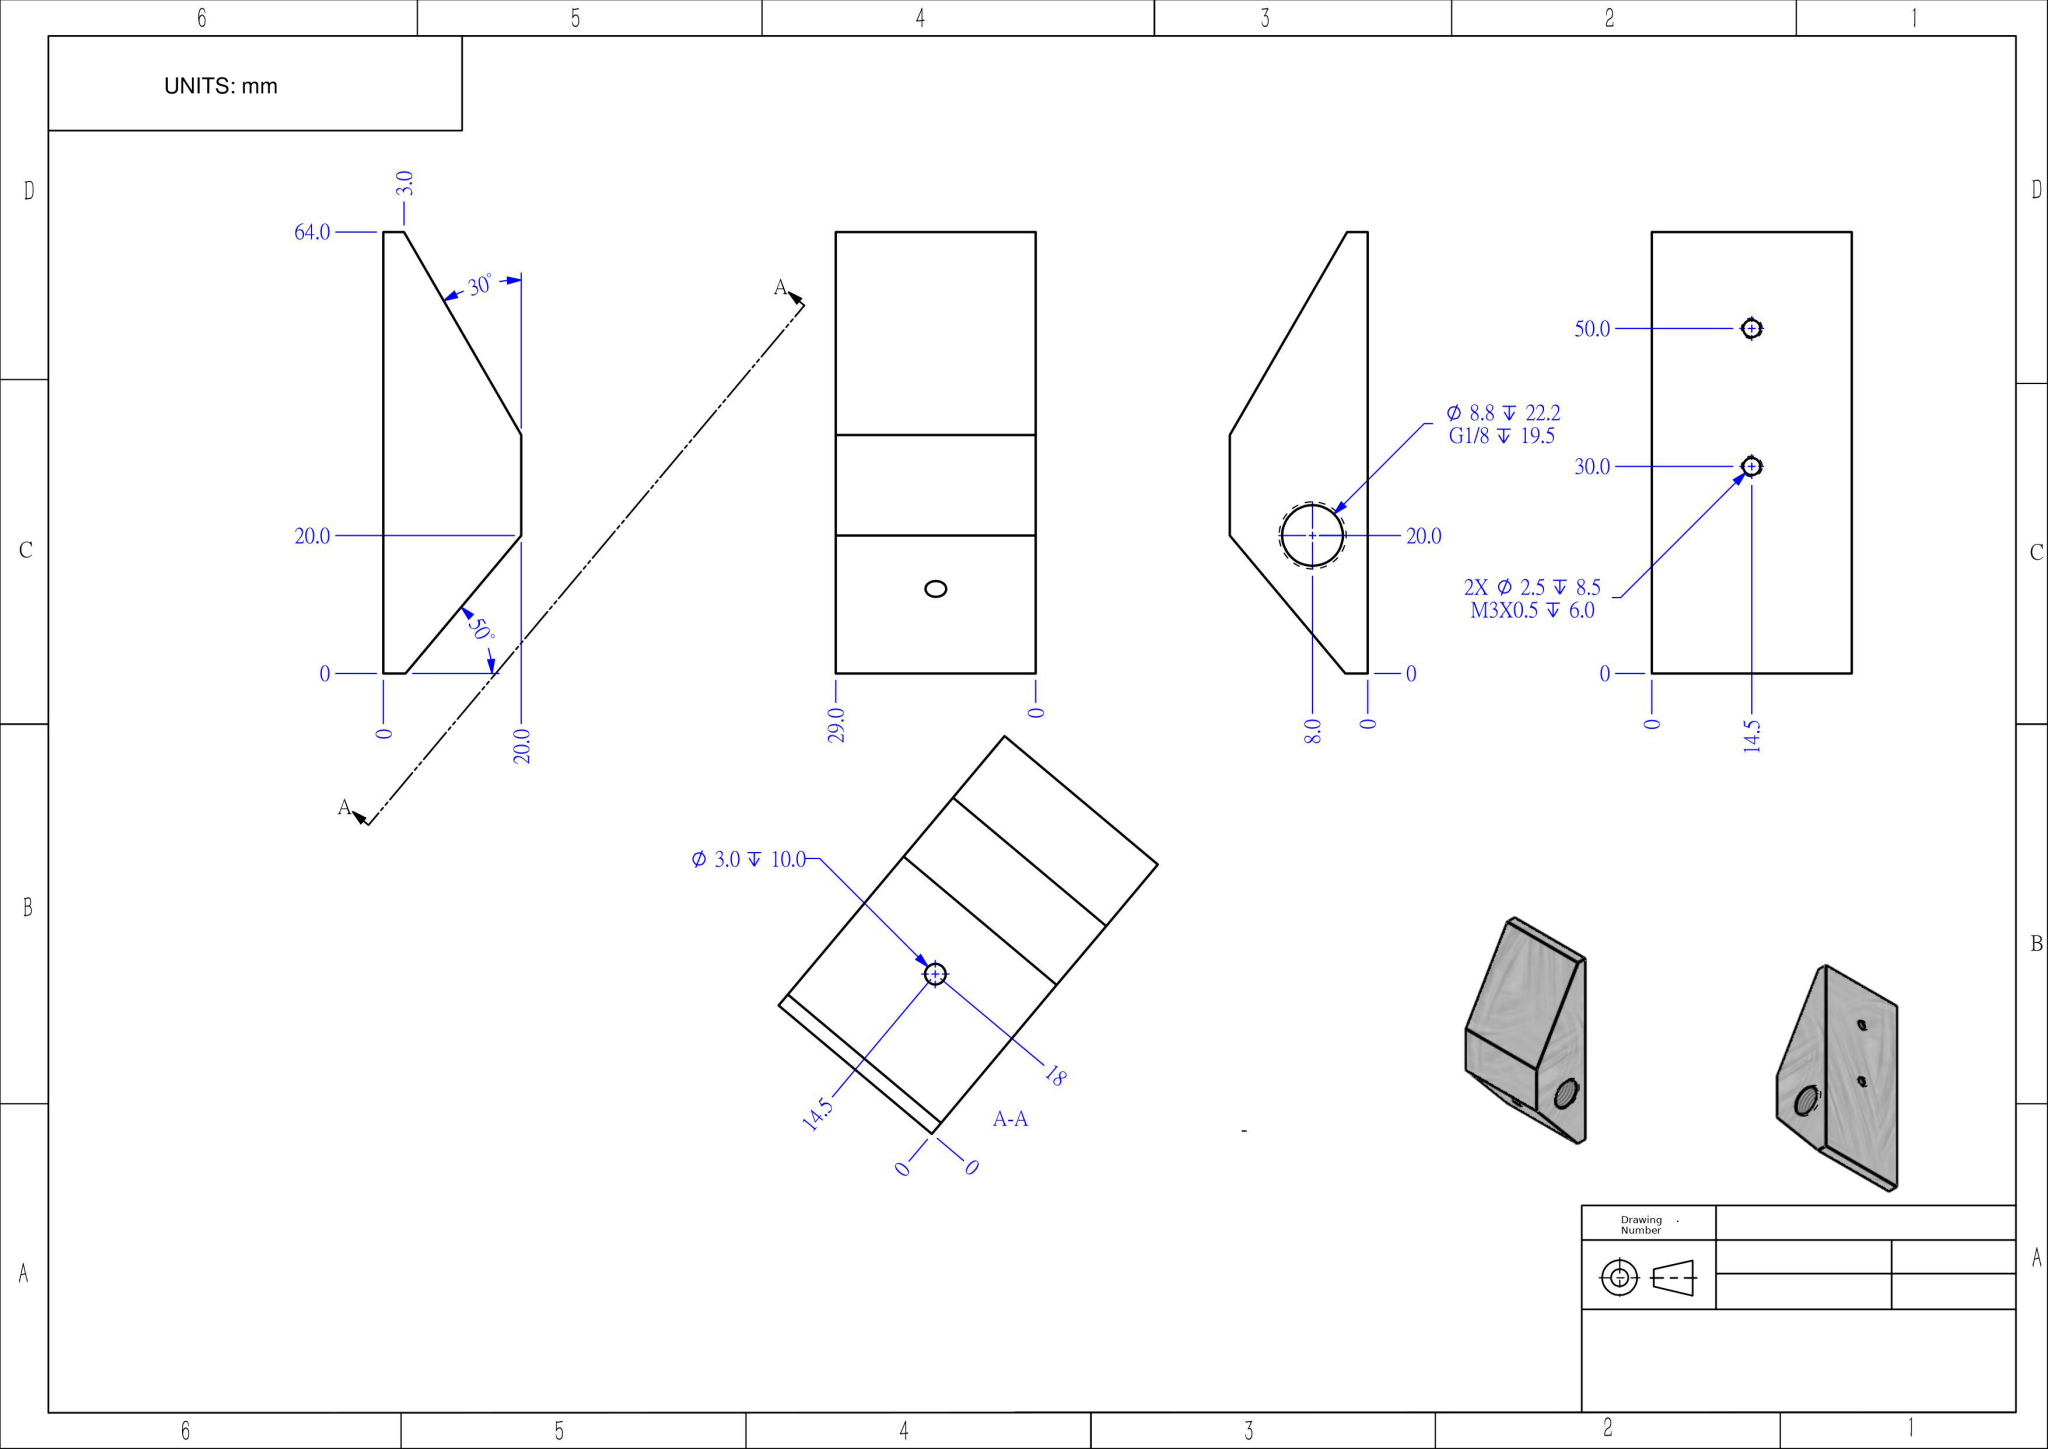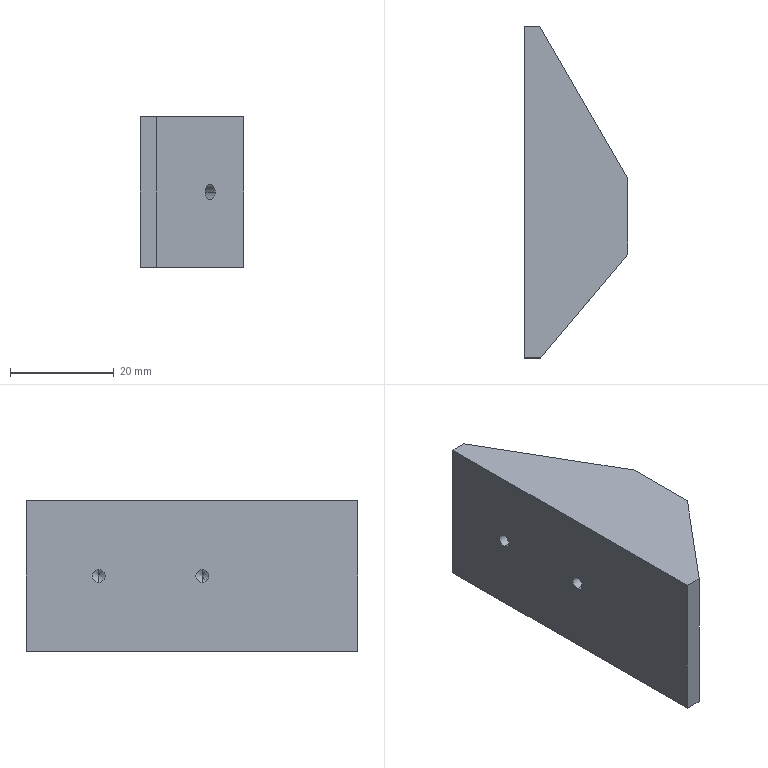Part | NX | mm | 1 solid | 22 faces | box 20 x 64 x 29 mm | volume 23467 mm3 | cylinder 8 | plane 8 | cone 6 | commonest cylinder face diameters 2.5 x4 8.8 x2 3 x2
STEP:
#1=COLOUR_RGB('',1.,1.,1.);
#2=FILL_AREA_STYLE_COLOUR('',#1);
#3=FILL_AREA_STYLE('',(#2));
#4=SURFACE_STYLE_FILL_AREA(#3);
#5=SURFACE_SIDE_STYLE('',(#4));
#6=SURFACE_STYLE_USAGE(.BOTH.,#5);
#7=PRESENTATION_STYLE_ASSIGNMENT((#6));
#8=CARTESIAN_POINT('',(-1.5,-2.,13.25));
#9=VERTEX_POINT('',#8);
#10=CARTESIAN_POINT('',(-10.,-2.,13.25));
#11=VERTEX_POINT('',#10);
#12=CARTESIAN_POINT('',(-10.,-2.,13.25));
#13=DIRECTION('',(-1.,0.,0.));
#14=VECTOR('',#13,1000.);
#15=LINE('',#12,#14);
#16=EDGE_CURVE('',#9,#11,#15,.T.);
#17=ORIENTED_EDGE('',*,*,#16,.F.);
#18=CARTESIAN_POINT('',(-1.5,-2.,15.75));
#19=VERTEX_POINT('',#18);
#20=CARTESIAN_POINT('',(-1.5,-2.,14.5));
#21=DIRECTION('',(-1.,0.,0.));
#22=DIRECTION('',(0.,0.,1.));
#23=AXIS2_PLACEMENT_3D('',#20,#21,#22);
#24=CIRCLE('',#23,1.25);
#25=EDGE_CURVE('',#19,#9,#24,.T.);
#26=ORIENTED_EDGE('',*,*,#25,.F.);
#27=CARTESIAN_POINT('',(-10.,-2.,15.75));
#28=VERTEX_POINT('',#27);
#29=CARTESIAN_POINT('',(-10.,-2.,15.75));
#30=DIRECTION('',(-1.,0.,0.));
#31=VECTOR('',#30,1000.);
#32=LINE('',#29,#31);
#33=EDGE_CURVE('',#19,#28,#32,.T.);
#34=ORIENTED_EDGE('',*,*,#33,.T.);
#35=CARTESIAN_POINT('',(-10.,-2.,14.5));
#36=DIRECTION('',(-1.,0.,0.));
#37=DIRECTION('',(0.,0.,1.));
#38=AXIS2_PLACEMENT_3D('',#35,#36,#37);
#39=CIRCLE('',#38,1.25);
#40=EDGE_CURVE('',#28,#11,#39,.T.);
#41=ORIENTED_EDGE('',*,*,#40,.T.);
#42=EDGE_LOOP('',(#17,#26,#34,#41));
#43=FACE_OUTER_BOUND('',#42,.T.);
#44=CARTESIAN_POINT('',(-10.,-2.,14.5));
#45=DIRECTION('',(-1.,0.,0.));
#46=DIRECTION('',(0.,0.,1.));
#47=AXIS2_PLACEMENT_3D('',#44,#45,#46);
#48=CYLINDRICAL_SURFACE('',#47,1.25);
#49=ADVANCED_FACE('',(#43),#48,.F.);
#50=STYLED_ITEM('',(#7),#49);
#51=(LENGTH_UNIT()NAMED_UNIT(*)SI_UNIT(.MILLI.,.METRE.));
#52=UNCERTAINTY_MEASURE_WITH_UNIT(LENGTH_MEASURE(0.00001),#51,'','');
#53=(NAMED_UNIT(*)PLANE_ANGLE_UNIT()SI_UNIT($,.RADIAN.));
#54=(NAMED_UNIT(*)SI_UNIT($,.STERADIAN.)SOLID_ANGLE_UNIT());
#55=(GEOMETRIC_REPRESENTATION_CONTEXT(3)GLOBAL_UNCERTAINTY_ASSIGNED_CONTEXT((#52))GLOBAL_UNIT_ASSIGNED_CONTEXT((#51,#53,#54))REPRESENTATION_CONTEXT('',''));
#56=MECHANICAL_DESIGN_GEOMETRIC_PRESENTATION_REPRESENTATION('',(#50),#55);
#57=COLOUR_RGB('',1.,1.,1.);
#58=FILL_AREA_STYLE_COLOUR('',#57);
#59=FILL_AREA_STYLE('',(#58));
#60=SURFACE_STYLE_FILL_AREA(#59);
#61=SURFACE_SIDE_STYLE('',(#60));
#62=SURFACE_STYLE_USAGE(.BOTH.,#61);
#63=PRESENTATION_STYLE_ASSIGNMENT((#62));
#64=CARTESIAN_POINT('',(2.4,-12.,22.177));
#65=VERTEX_POINT('',#64);
#66=CARTESIAN_POINT('',(2.4,-12.,-0.));
#67=VERTEX_POINT('',#66);
#68=CARTESIAN_POINT('',(2.4,-12.,0.));
#69=DIRECTION('',(0.,0.,-1.));
#70=VECTOR('',#69,1000.);
#71=LINE('',#68,#70);
#72=EDGE_CURVE('',#65,#67,#71,.T.);
#73=ORIENTED_EDGE('',*,*,#72,.F.);
#74=CARTESIAN_POINT('',(-6.4,-12.,22.177));
#75=VERTEX_POINT('',#74);
#76=CARTESIAN_POINT('',(-2.,-12.,22.177));
#77=DIRECTION('',(0.,0.,-1.));
#78=DIRECTION('',(-1.,0.,0.));
#79=AXIS2_PLACEMENT_3D('',#76,#77,#78);
#80=CIRCLE('',#79,4.4);
#81=EDGE_CURVE('',#75,#65,#80,.T.);
#82=ORIENTED_EDGE('',*,*,#81,.F.);
#83=CARTESIAN_POINT('',(-6.4,-12.,-0.));
#84=VERTEX_POINT('',#83);
#85=CARTESIAN_POINT('',(-6.4,-12.,0.));
#86=DIRECTION('',(0.,0.,-1.));
#87=VECTOR('',#86,1000.);
#88=LINE('',#85,#87);
#89=EDGE_CURVE('',#75,#84,#88,.T.);
#90=ORIENTED_EDGE('',*,*,#89,.T.);
#91=CARTESIAN_POINT('',(-2.,-12.,-0.));
#92=DIRECTION('',(0.,0.,-1.));
#93=DIRECTION('',(-1.,0.,0.));
#94=AXIS2_PLACEMENT_3D('',#91,#92,#93);
#95=CIRCLE('',#94,4.4);
#96=EDGE_CURVE('',#84,#67,#95,.T.);
#97=ORIENTED_EDGE('',*,*,#96,.T.);
#98=EDGE_LOOP('',(#73,#82,#90,#97));
#99=FACE_OUTER_BOUND('',#98,.T.);
#100=CARTESIAN_POINT('',(-2.,-12.,0.));
#101=DIRECTION('',(0.,0.,-1.));
#102=DIRECTION('',(-1.,0.,0.));
#103=AXIS2_PLACEMENT_3D('',#100,#101,#102);
#104=CYLINDRICAL_SURFACE('',#103,4.4);
#105=ADVANCED_FACE('',(#99),#104,.F.);
#106=STYLED_ITEM('',(#63),#105);
#107=(LENGTH_UNIT()NAMED_UNIT(*)SI_UNIT(.MILLI.,.METRE.));
#108=UNCERTAINTY_MEASURE_WITH_UNIT(LENGTH_MEASURE(0.00001),#107,'','');
#109=(NAMED_UNIT(*)PLANE_ANGLE_UNIT()SI_UNIT($,.RADIAN.));
#110=(NAMED_UNIT(*)SI_UNIT($,.STERADIAN.)SOLID_ANGLE_UNIT());
#111=(GEOMETRIC_REPRESENTATION_CONTEXT(3)GLOBAL_UNCERTAINTY_ASSIGNED_CONTEXT((#108))GLOBAL_UNIT_ASSIGNED_CONTEXT((#107,#109,#110))REPRESENTATION_CONTEXT('',''));
#112=MECHANICAL_DESIGN_GEOMETRIC_PRESENTATION_REPRESENTATION('',(#106),#111);
#113=COLOUR_RGB('',1.,1.,1.);
#114=FILL_AREA_STYLE_COLOUR('',#113);
#115=FILL_AREA_STYLE('',(#114));
#116=SURFACE_STYLE_FILL_AREA(#115);
#117=SURFACE_SIDE_STYLE('',(#116));
#118=SURFACE_STYLE_USAGE(.BOTH.,#117);
#119=PRESENTATION_STYLE_ASSIGNMENT((#118));
#120=CARTESIAN_POINT('',(-1.5,18.,13.25));
#121=VERTEX_POINT('',#120);
#122=CARTESIAN_POINT('',(-1.5,18.,15.75));
#123=VERTEX_POINT('',#122);
#124=CARTESIAN_POINT('',(-1.5,18.,14.5));
#125=DIRECTION('',(-1.,0.,0.));
#126=DIRECTION('',(0.,0.,1.));
#127=AXIS2_PLACEMENT_3D('',#124,#125,#126);
#128=CIRCLE('',#127,1.25);
#129=EDGE_CURVE('',#121,#123,#128,.T.);
#130=ORIENTED_EDGE('',*,*,#129,.F.);
#131=CARTESIAN_POINT('',(-10.,18.,13.25));
#132=VERTEX_POINT('',#131);
#133=CARTESIAN_POINT('',(-10.,18.,13.25));
#134=DIRECTION('',(-1.,0.,0.));
#135=VECTOR('',#134,1000.);
#136=LINE('',#133,#135);
#137=EDGE_CURVE('',#121,#132,#136,.T.);
#138=ORIENTED_EDGE('',*,*,#137,.T.);
#139=CARTESIAN_POINT('',(-10.,18.,15.75));
#140=VERTEX_POINT('',#139);
#141=CARTESIAN_POINT('',(-10.,18.,14.5));
#142=DIRECTION('',(-1.,0.,0.));
#143=DIRECTION('',(0.,0.,1.));
#144=AXIS2_PLACEMENT_3D('',#141,#142,#143);
#145=CIRCLE('',#144,1.25);
#146=EDGE_CURVE('',#132,#140,#145,.T.);
#147=ORIENTED_EDGE('',*,*,#146,.T.);
#148=CARTESIAN_POINT('',(-10.,18.,15.75));
#149=DIRECTION('',(-1.,0.,0.));
#150=VECTOR('',#149,1000.);
#151=LINE('',#148,#150);
#152=EDGE_CURVE('',#123,#140,#151,.T.);
#153=ORIENTED_EDGE('',*,*,#152,.F.);
#154=EDGE_LOOP('',(#130,#138,#147,#153));
#155=FACE_OUTER_BOUND('',#154,.T.);
#156=CARTESIAN_POINT('',(-10.,18.,14.5));
#157=DIRECTION('',(-1.,0.,0.));
#158=DIRECTION('',(0.,0.,1.));
#159=AXIS2_PLACEMENT_3D('',#156,#157,#158);
#160=CYLINDRICAL_SURFACE('',#159,1.25);
#161=ADVANCED_FACE('',(#155),#160,.F.);
#162=CARTESIAN_POINT('',(-0.7489,18.,14.5));
#163=VERTEX_POINT('',#162);
#164=CARTESIAN_POINT('',(-1.5,18.,15.75));
#165=DIRECTION('',(-0.515,0.,0.8572));
#166=VECTOR('',#165,1000.);
#167=LINE('',#164,#166);
#168=EDGE_CURVE('',#163,#123,#167,.T.);
#169=ORIENTED_EDGE('',*,*,#168,.F.);
#170=CARTESIAN_POINT('',(-1.5,18.,13.25));
#171=DIRECTION('',(-0.515,0.,-0.8572));
#172=VECTOR('',#171,1000.);
#173=LINE('',#170,#172);
#174=EDGE_CURVE('',#163,#121,#173,.T.);
#175=ORIENTED_EDGE('',*,*,#174,.T.);
#176=ORIENTED_EDGE('',*,*,#129,.T.);
#177=EDGE_LOOP('',(#169,#175,#176));
#178=FACE_OUTER_BOUND('',#177,.T.);
#179=CARTESIAN_POINT('',(-1.5,18.,14.5));
#180=DIRECTION('',(-1.,0.,0.));
#181=DIRECTION('',(0.,0.,1.));
#182=AXIS2_PLACEMENT_3D('',#179,#180,#181);
#183=CONICAL_SURFACE('',#182,1.25,1.03);
#184=ADVANCED_FACE('',(#178),#183,.F.);
#185=CARTESIAN_POINT('',(-1.5,-2.,14.5));
#186=DIRECTION('',(-1.,0.,0.));
#187=DIRECTION('',(0.,0.,1.));
#188=AXIS2_PLACEMENT_3D('',#185,#186,#187);
#189=CIRCLE('',#188,1.25);
#190=EDGE_CURVE('',#9,#19,#189,.T.);
#191=ORIENTED_EDGE('',*,*,#190,.F.);
#192=ORIENTED_EDGE('',*,*,#16,.T.);
#193=CARTESIAN_POINT('',(-10.,-2.,14.5));
#194=DIRECTION('',(-1.,0.,0.));
#195=DIRECTION('',(0.,0.,1.));
#196=AXIS2_PLACEMENT_3D('',#193,#194,#195);
#197=CIRCLE('',#196,1.25);
#198=EDGE_CURVE('',#11,#28,#197,.T.);
#199=ORIENTED_EDGE('',*,*,#198,.T.);
#200=ORIENTED_EDGE('',*,*,#33,.F.);
#201=EDGE_LOOP('',(#191,#192,#199,#200));
#202=FACE_OUTER_BOUND('',#201,.T.);
#203=CARTESIAN_POINT('',(-10.,-2.,14.5));
#204=DIRECTION('',(-1.,0.,0.));
#205=DIRECTION('',(0.,0.,1.));
#206=AXIS2_PLACEMENT_3D('',#203,#204,#205);
#207=CYLINDRICAL_SURFACE('',#206,1.25);
#208=ADVANCED_FACE('',(#202),#207,.F.);
#209=CARTESIAN_POINT('',(-0.7489,-2.,14.5));
#210=VERTEX_POINT('',#209);
#211=CARTESIAN_POINT('',(-1.5,-2.,15.75));
#212=DIRECTION('',(-0.515,0.,0.8572));
#213=VECTOR('',#212,1000.);
#214=LINE('',#211,#213);
#215=EDGE_CURVE('',#210,#19,#214,.T.);
#216=ORIENTED_EDGE('',*,*,#215,.F.);
#217=CARTESIAN_POINT('',(-1.5,-2.,13.25));
#218=DIRECTION('',(-0.515,0.,-0.8572));
#219=VECTOR('',#218,1000.);
#220=LINE('',#217,#219);
#221=EDGE_CURVE('',#210,#9,#220,.T.);
#222=ORIENTED_EDGE('',*,*,#221,.T.);
#223=ORIENTED_EDGE('',*,*,#190,.T.);
#224=EDGE_LOOP('',(#216,#222,#223));
#225=FACE_OUTER_BOUND('',#224,.T.);
#226=CARTESIAN_POINT('',(-1.5,-2.,14.5));
#227=DIRECTION('',(-1.,0.,0.));
#228=DIRECTION('',(0.,0.,1.));
#229=AXIS2_PLACEMENT_3D('',#226,#227,#228);
#230=CONICAL_SURFACE('',#229,1.25,1.03);
#231=ADVANCED_FACE('',(#225),#230,.F.);
#232=CARTESIAN_POINT('',(-2.,-12.,24.821));
#233=VERTEX_POINT('',#232);
#234=CARTESIAN_POINT('',(-6.4,-12.,22.177));
#235=DIRECTION('',(-0.8572,0.,-0.515));
#236=VECTOR('',#235,1000.);
#237=LINE('',#234,#236);
#238=EDGE_CURVE('',#233,#75,#237,.T.);
#239=ORIENTED_EDGE('',*,*,#238,.F.);
#240=CARTESIAN_POINT('',(2.4,-12.,22.177));
#241=DIRECTION('',(0.8572,0.,-0.515));
#242=VECTOR('',#241,1000.);
#243=LINE('',#240,#242);
#244=EDGE_CURVE('',#233,#65,#243,.T.);
#245=ORIENTED_EDGE('',*,*,#244,.T.);
#246=CARTESIAN_POINT('',(-2.,-12.,22.177));
#247=DIRECTION('',(0.,0.,-1.));
#248=DIRECTION('',(-1.,0.,0.));
#249=AXIS2_PLACEMENT_3D('',#246,#247,#248);
#250=CIRCLE('',#249,4.4);
#251=EDGE_CURVE('',#65,#75,#250,.T.);
#252=ORIENTED_EDGE('',*,*,#251,.T.);
#253=EDGE_LOOP('',(#239,#245,#252));
#254=FACE_OUTER_BOUND('',#253,.T.);
#255=CARTESIAN_POINT('',(-2.,-12.,22.177));
#256=DIRECTION('',(0.,0.,-1.));
#257=DIRECTION('',(-1.,0.,0.));
#258=AXIS2_PLACEMENT_3D('',#255,#256,#257);
#259=CONICAL_SURFACE('',#258,4.4,1.03);
#260=ADVANCED_FACE('',(#254),#259,.F.);
#261=CARTESIAN_POINT('',(0.7251,-15.455,14.5));
#262=VERTEX_POINT('',#261);
#263=CARTESIAN_POINT('',(-2.935,-16.299,14.5));
#264=VERTEX_POINT('',#263);
#265=CARTESIAN_POINT('',(0.7251,-15.455,14.5));
#266=CARTESIAN_POINT('',(0.7251,-15.455,14.387));
#267=CARTESIAN_POINT('',(0.715,-15.463,14.276));
#268=CARTESIAN_POINT('',(0.6748,-15.494,14.058));
#269=CARTESIAN_POINT('',(0.6441,-15.517,13.95));
#270=CARTESIAN_POINT('',(0.5241,-15.605,13.649));
#271=CARTESIAN_POINT('',(0.4035,-15.69,13.471));
#272=CARTESIAN_POINT('',(0.1742,-15.826,13.267));
#273=CARTESIAN_POINT('',(0.08867,-15.874,13.208));
#274=CARTESIAN_POINT('',(-0.09207,-15.966,13.114));
#275=CARTESIAN_POINT('',(-0.1889,-16.011,13.077));
#276=CARTESIAN_POINT('',(-0.492,-16.139,12.999));
#277=CARTESIAN_POINT('',(-0.708,-16.212,12.989));
#278=CARTESIAN_POINT('',(-1.14,-16.321,13.033));
#279=CARTESIAN_POINT('',(-1.359,-16.358,13.087));
#280=CARTESIAN_POINT('',(-1.777,-16.399,13.241));
#281=CARTESIAN_POINT('',(-1.981,-16.404,13.341));
#282=CARTESIAN_POINT('',(-2.357,-16.39,13.581));
#283=CARTESIAN_POINT('',(-2.531,-16.37,13.72));
#284=CARTESIAN_POINT('',(-2.75,-16.336,13.977));
#285=CARTESIAN_POINT('',(-2.814,-16.324,14.071));
#286=CARTESIAN_POINT('',(-2.884,-16.31,14.225));
#287=CARTESIAN_POINT('',(-2.903,-16.306,14.277));
#288=CARTESIAN_POINT('',(-2.928,-16.301,14.386));
#289=CARTESIAN_POINT('',(-2.935,-16.299,14.444));
#290=CARTESIAN_POINT('',(-2.935,-16.299,14.5));
#291=B_SPLINE_CURVE_WITH_KNOTS('',3,(#265,#266,#267,#268,#269,#270,#271,#272,#273,#274,#275,#276,#277,#278,#279,#280,#281,#282,#283,#284,#285,#286,#287,#288,#289,#290),.UNSPECIFIED.,.F.,.F.,(4,2,2,2,2,2,2,2,2,2,2,2,4),(0.,0.0003351,0.0006703,0.001341,0.001676,0.002011,0.002681,0.003351,0.004022,0.004692,0.005027,0.005194,0.005362),.UNSPECIFIED.);
#292=EDGE_CURVE('',#262,#264,#291,.T.);
#293=ORIENTED_EDGE('',*,*,#292,.F.);
#294=CARTESIAN_POINT('',(-2.935,-16.299,14.5));
#295=CARTESIAN_POINT('',(-2.935,-16.299,14.612));
#296=CARTESIAN_POINT('',(-2.907,-16.306,14.725));
#297=CARTESIAN_POINT('',(-2.814,-16.324,14.928));
#298=CARTESIAN_POINT('',(-2.75,-16.336,15.022));
#299=CARTESIAN_POINT('',(-2.534,-16.37,15.278));
#300=CARTESIAN_POINT('',(-2.356,-16.39,15.42));
#301=CARTESIAN_POINT('',(-1.98,-16.404,15.66));
#302=CARTESIAN_POINT('',(-1.778,-16.399,15.759));
#303=CARTESIAN_POINT('',(-1.358,-16.358,15.913));
#304=CARTESIAN_POINT('',(-1.145,-16.322,15.966));
#305=CARTESIAN_POINT('',(-0.8213,-16.241,16.));
#306=CARTESIAN_POINT('',(-0.7117,-16.209,16.003));
#307=CARTESIAN_POINT('',(-0.4994,-16.138,15.991));
#308=CARTESIAN_POINT('',(-0.3956,-16.099,15.976));
#309=CARTESIAN_POINT('',(-0.09186,-15.971,15.898));
#310=CARTESIAN_POINT('',(0.09184,-15.875,15.805));
#311=CARTESIAN_POINT('',(0.3245,-15.737,15.599));
#312=CARTESIAN_POINT('',(0.3927,-15.693,15.522));
#313=CARTESIAN_POINT('',(0.5117,-15.613,15.35));
#314=CARTESIAN_POINT('',(0.5627,-15.577,15.253));
#315=CARTESIAN_POINT('',(0.6836,-15.488,14.952));
#316=CARTESIAN_POINT('',(0.7251,-15.455,14.726));
#317=CARTESIAN_POINT('',(0.7251,-15.455,14.5));
#318=B_SPLINE_CURVE_WITH_KNOTS('',3,(#294,#295,#296,#297,#298,#299,#300,#301,#302,#303,#304,#305,#306,#307,#308,#309,#310,#311,#312,#313,#314,#315,#316,#317),.UNSPECIFIED.,.F.,.F.,(4,2,2,2,2,2,2,2,2,2,2,4),(0.005362,0.005697,0.006032,0.006701,0.007371,0.00804,0.008375,0.00871,0.00938,0.009714,0.01005,0.01072),.UNSPECIFIED.);
#319=EDGE_CURVE('',#264,#262,#318,.T.);
#320=ORIENTED_EDGE('',*,*,#319,.F.);
#321=EDGE_LOOP('',(#293,#320));
#322=FACE_BOUND('',#321,.T.);
#323=ORIENTED_EDGE('',*,*,#251,.F.);
#324=ORIENTED_EDGE('',*,*,#72,.T.);
#325=CARTESIAN_POINT('',(-2.,-12.,-0.));
#326=DIRECTION('',(0.,0.,-1.));
#327=DIRECTION('',(-1.,0.,0.));
#328=AXIS2_PLACEMENT_3D('',#325,#326,#327);
#329=CIRCLE('',#328,4.4);
#330=EDGE_CURVE('',#67,#84,#329,.T.);
#331=ORIENTED_EDGE('',*,*,#330,.T.);
#332=ORIENTED_EDGE('',*,*,#89,.F.);
#333=EDGE_LOOP('',(#323,#324,#331,#332));
#334=FACE_OUTER_BOUND('',#333,.T.);
#335=CARTESIAN_POINT('',(-2.,-12.,0.));
#336=DIRECTION('',(0.,0.,-1.));
#337=DIRECTION('',(-1.,0.,0.));
#338=AXIS2_PLACEMENT_3D('',#335,#336,#337);
#339=CYLINDRICAL_SURFACE('',#338,4.4);
#340=ADVANCED_FACE('',(#322,#334),#339,.F.);
#341=ORIENTED_EDGE('',*,*,#292,.T.);
#342=CARTESIAN_POINT('',(2.538,-20.892,14.5));
#343=VERTEX_POINT('',#342);
#344=CARTESIAN_POINT('',(2.538,-20.892,14.5));
#345=DIRECTION('',(0.766,-0.6428,0.));
#346=VECTOR('',#345,1000.);
#347=LINE('',#344,#346);
#348=EDGE_CURVE('',#264,#343,#347,.T.);
#349=ORIENTED_EDGE('',*,*,#348,.T.);
#350=CARTESIAN_POINT('',(4.467,-18.594,14.5));
#351=VERTEX_POINT('',#350);
#352=CARTESIAN_POINT('',(3.503,-19.743,14.5));
#353=DIRECTION('',(0.766,-0.6428,0.));
#354=DIRECTION('',(0.6428,0.766,0.));
#355=AXIS2_PLACEMENT_3D('',#352,#353,#354);
#356=CIRCLE('',#355,1.5);
#357=EDGE_CURVE('',#343,#351,#356,.T.);
#358=ORIENTED_EDGE('',*,*,#357,.T.);
#359=CARTESIAN_POINT('',(4.467,-18.594,14.5));
#360=DIRECTION('',(0.766,-0.6428,0.));
#361=VECTOR('',#360,1000.);
#362=LINE('',#359,#361);
#363=EDGE_CURVE('',#262,#351,#362,.T.);
#364=ORIENTED_EDGE('',*,*,#363,.F.);
#365=EDGE_LOOP('',(#341,#349,#358,#364));
#366=FACE_OUTER_BOUND('',#365,.T.);
#367=CARTESIAN_POINT('',(3.503,-19.743,14.5));
#368=DIRECTION('',(0.766,-0.6428,0.));
#369=DIRECTION('',(0.6428,0.766,0.));
#370=AXIS2_PLACEMENT_3D('',#367,#368,#369);
#371=CYLINDRICAL_SURFACE('',#370,1.5);
#372=ADVANCED_FACE('',(#366),#371,.F.);
#373=CARTESIAN_POINT('',(10.,-12.,0.));
#374=VERTEX_POINT('',#373);
#375=CARTESIAN_POINT('',(10.,2.555,0.));
#376=VERTEX_POINT('',#375);
#377=CARTESIAN_POINT('',(10.,-32.,0.));
#378=DIRECTION('',(0.,1.,0.));
#379=VECTOR('',#378,1000.);
#380=LINE('',#377,#379);
#381=EDGE_CURVE('',#374,#376,#380,.T.);
#382=ORIENTED_EDGE('',*,*,#381,.T.);
#383=CARTESIAN_POINT('',(10.,2.555,29.));
#384=VERTEX_POINT('',#383);
#385=CARTESIAN_POINT('',(10.,2.555,0.));
#386=DIRECTION('',(0.,0.,1.));
#387=VECTOR('',#386,1000.);
#388=LINE('',#385,#387);
#389=EDGE_CURVE('',#376,#384,#388,.T.);
#390=ORIENTED_EDGE('',*,*,#389,.T.);
#391=CARTESIAN_POINT('',(10.,-12.,29.));
#392=VERTEX_POINT('',#391);
#393=CARTESIAN_POINT('',(10.,-32.,29.));
#394=DIRECTION('',(0.,1.,0.));
#395=VECTOR('',#394,1000.);
#396=LINE('',#393,#395);
#397=EDGE_CURVE('',#392,#384,#396,.T.);
#398=ORIENTED_EDGE('',*,*,#397,.F.);
#399=CARTESIAN_POINT('',(10.,-12.,0.));
#400=DIRECTION('',(0.,0.,1.));
#401=VECTOR('',#400,1000.);
#402=LINE('',#399,#401);
#403=EDGE_CURVE('',#374,#392,#402,.T.);
#404=ORIENTED_EDGE('',*,*,#403,.F.);
#405=EDGE_LOOP('',(#382,#390,#398,#404));
#406=FACE_OUTER_BOUND('',#405,.T.);
#407=CARTESIAN_POINT('',(10.,-32.,29.));
#408=DIRECTION('',(-1.,0.,0.));
#409=DIRECTION('',(0.,0.,1.));
#410=AXIS2_PLACEMENT_3D('',#407,#408,#409);
#411=PLANE('',#410);
#412=ADVANCED_FACE('',(#406),#411,.F.);
#413=CARTESIAN_POINT('',(-7.,32.,29.));
#414=VERTEX_POINT('',#413);
#415=CARTESIAN_POINT('',(-10.,32.,29.));
#416=VERTEX_POINT('',#415);
#417=CARTESIAN_POINT('',(-10.,32.,29.));
#418=DIRECTION('',(-1.,0.,0.));
#419=VECTOR('',#418,1000.);
#420=LINE('',#417,#419);
#421=EDGE_CURVE('',#414,#416,#420,.T.);
#422=ORIENTED_EDGE('',*,*,#421,.F.);
#423=CARTESIAN_POINT('',(-7.,32.,0.));
#424=VERTEX_POINT('',#423);
#425=CARTESIAN_POINT('',(-7.,32.,0.));
#426=DIRECTION('',(0.,0.,1.));
#427=VECTOR('',#426,1000.);
#428=LINE('',#425,#427);
#429=EDGE_CURVE('',#424,#414,#428,.T.);
#430=ORIENTED_EDGE('',*,*,#429,.F.);
#431=CARTESIAN_POINT('',(-10.,32.,0.));
#432=VERTEX_POINT('',#431);
#433=CARTESIAN_POINT('',(-10.,32.,0.));
#434=DIRECTION('',(-1.,0.,0.));
#435=VECTOR('',#434,1000.);
#436=LINE('',#433,#435);
#437=EDGE_CURVE('',#424,#432,#436,.T.);
#438=ORIENTED_EDGE('',*,*,#437,.T.);
#439=CARTESIAN_POINT('',(-10.,32.,29.));
#440=DIRECTION('',(0.,0.,-1.));
#441=VECTOR('',#440,1000.);
#442=LINE('',#439,#441);
#443=EDGE_CURVE('',#416,#432,#442,.T.);
#444=ORIENTED_EDGE('',*,*,#443,.F.);
#445=EDGE_LOOP('',(#422,#430,#438,#444));
#446=FACE_OUTER_BOUND('',#445,.T.);
#447=CARTESIAN_POINT('',(-10.,32.,29.));
#448=DIRECTION('',(0.,-1.,0.));
#449=DIRECTION('',(0.,0.,-1.));
#450=AXIS2_PLACEMENT_3D('',#447,#448,#449);
#451=PLANE('',#450);
#452=ADVANCED_FACE('',(#446),#451,.F.);
#453=CARTESIAN_POINT('',(-10.,18.,14.5));
#454=DIRECTION('',(-1.,0.,0.));
#455=DIRECTION('',(0.,0.,1.));
#456=AXIS2_PLACEMENT_3D('',#453,#454,#455);
#457=CIRCLE('',#456,1.25);
#458=EDGE_CURVE('',#140,#132,#457,.T.);
#459=ORIENTED_EDGE('',*,*,#458,.F.);
#460=ORIENTED_EDGE('',*,*,#146,.F.);
#461=EDGE_LOOP('',(#459,#460));
#462=FACE_BOUND('',#461,.T.);
#463=ORIENTED_EDGE('',*,*,#40,.F.);
#464=ORIENTED_EDGE('',*,*,#198,.F.);
#465=EDGE_LOOP('',(#463,#464));
#466=FACE_BOUND('',#465,.T.);
#467=CARTESIAN_POINT('',(-10.,-32.,0.));
#468=VERTEX_POINT('',#467);
#469=CARTESIAN_POINT('',(-10.,-32.,0.));
#470=DIRECTION('',(0.,-1.,0.));
#471=VECTOR('',#470,1000.);
#472=LINE('',#469,#471);
#473=EDGE_CURVE('',#432,#468,#472,.T.);
#474=ORIENTED_EDGE('',*,*,#473,.T.);
#475=CARTESIAN_POINT('',(-10.,-32.,29.));
#476=VERTEX_POINT('',#475);
#477=CARTESIAN_POINT('',(-10.,-32.,29.));
#478=DIRECTION('',(0.,0.,-1.));
#479=VECTOR('',#478,1000.);
#480=LINE('',#477,#479);
#481=EDGE_CURVE('',#476,#468,#480,.T.);
#482=ORIENTED_EDGE('',*,*,#481,.F.);
#483=CARTESIAN_POINT('',(-10.,-32.,29.));
#484=DIRECTION('',(0.,-1.,0.));
#485=VECTOR('',#484,1000.);
#486=LINE('',#483,#485);
#487=EDGE_CURVE('',#416,#476,#486,.T.);
#488=ORIENTED_EDGE('',*,*,#487,.F.);
#489=ORIENTED_EDGE('',*,*,#443,.T.);
#490=EDGE_LOOP('',(#474,#482,#488,#489));
#491=FACE_OUTER_BOUND('',#490,.T.);
#492=CARTESIAN_POINT('',(-10.,-32.,29.));
#493=DIRECTION('',(1.,0.,0.));
#494=DIRECTION('',(0.,0.,-1.));
#495=AXIS2_PLACEMENT_3D('',#492,#493,#494);
#496=PLANE('',#495);
#497=ADVANCED_FACE('',(#462,#466,#491),#496,.F.);
#498=CARTESIAN_POINT('',(-6.782,-32.,0.));
#499=VERTEX_POINT('',#498);
#500=CARTESIAN_POINT('',(-10.,-32.,0.));
#501=DIRECTION('',(1.,0.,0.));
#502=VECTOR('',#501,1000.);
#503=LINE('',#500,#502);
#504=EDGE_CURVE('',#468,#499,#503,.T.);
#505=ORIENTED_EDGE('',*,*,#504,.T.);
#506=CARTESIAN_POINT('',(-6.782,-32.,29.));
#507=VERTEX_POINT('',#506);
#508=CARTESIAN_POINT('',(-6.782,-32.,0.));
#509=DIRECTION('',(0.,0.,1.));
#510=VECTOR('',#509,1000.);
#511=LINE('',#508,#510);
#512=EDGE_CURVE('',#499,#507,#511,.T.);
#513=ORIENTED_EDGE('',*,*,#512,.T.);
#514=CARTESIAN_POINT('',(-10.,-32.,29.));
#515=DIRECTION('',(1.,0.,0.));
#516=VECTOR('',#515,1000.);
#517=LINE('',#514,#516);
#518=EDGE_CURVE('',#476,#507,#517,.T.);
#519=ORIENTED_EDGE('',*,*,#518,.F.);
#520=ORIENTED_EDGE('',*,*,#481,.T.);
#521=EDGE_LOOP('',(#505,#513,#519,#520));
#522=FACE_OUTER_BOUND('',#521,.T.);
#523=CARTESIAN_POINT('',(-10.,-32.,29.));
#524=DIRECTION('',(0.,1.,0.));
#525=DIRECTION('',(0.,0.,1.));
#526=AXIS2_PLACEMENT_3D('',#523,#524,#525);
#527=PLANE('',#526);
#528=ADVANCED_FACE('',(#522),#527,.F.);
#529=ORIENTED_EDGE('',*,*,#397,.T.);
#530=CARTESIAN_POINT('',(-7.,32.,29.));
#531=DIRECTION('',(0.5,-0.866,0.));
#532=VECTOR('',#531,1000.);
#533=LINE('',#530,#532);
#534=EDGE_CURVE('',#414,#384,#533,.T.);
#535=ORIENTED_EDGE('',*,*,#534,.F.);
#536=ORIENTED_EDGE('',*,*,#421,.T.);
#537=ORIENTED_EDGE('',*,*,#487,.T.);
#538=ORIENTED_EDGE('',*,*,#518,.T.);
#539=CARTESIAN_POINT('',(10.,-12.,29.));
#540=DIRECTION('',(-0.6428,-0.766,0.));
#541=VECTOR('',#540,1000.);
#542=LINE('',#539,#541);
#543=EDGE_CURVE('',#392,#507,#542,.T.);
#544=ORIENTED_EDGE('',*,*,#543,.F.);
#545=EDGE_LOOP('',(#529,#535,#536,#537,#538,#544));
#546=FACE_OUTER_BOUND('',#545,.T.);
#547=CARTESIAN_POINT('',(0.,0.,29.));
#548=DIRECTION('',(0.,0.,-1.));
#549=DIRECTION('',(-1.,0.,0.));
#550=AXIS2_PLACEMENT_3D('',#547,#548,#549);
#551=PLANE('',#550);
#552=ADVANCED_FACE('',(#546),#551,.F.);
#553=ORIENTED_EDGE('',*,*,#96,.F.);
#554=ORIENTED_EDGE('',*,*,#330,.F.);
#555=EDGE_LOOP('',(#553,#554));
#556=FACE_BOUND('',#555,.T.);
#557=CARTESIAN_POINT('',(-7.,32.,0.));
#558=DIRECTION('',(0.5,-0.866,0.));
#559=VECTOR('',#558,1000.);
#560=LINE('',#557,#559);
#561=EDGE_CURVE('',#424,#376,#560,.T.);
#562=ORIENTED_EDGE('',*,*,#561,.T.);
#563=ORIENTED_EDGE('',*,*,#381,.F.);
#564=CARTESIAN_POINT('',(10.,-12.,0.));
#565=DIRECTION('',(-0.6428,-0.766,0.));
#566=VECTOR('',#565,1000.);
#567=LINE('',#564,#566);
#568=EDGE_CURVE('',#374,#499,#567,.T.);
#569=ORIENTED_EDGE('',*,*,#568,.T.);
#570=ORIENTED_EDGE('',*,*,#504,.F.);
#571=ORIENTED_EDGE('',*,*,#473,.F.);
#572=ORIENTED_EDGE('',*,*,#437,.F.);
#573=EDGE_LOOP('',(#562,#563,#569,#570,#571,#572));
#574=FACE_OUTER_BOUND('',#573,.T.);
#575=CARTESIAN_POINT('',(0.,0.,0.));
#576=DIRECTION('',(0.,0.,-1.));
#577=DIRECTION('',(-1.,0.,0.));
#578=AXIS2_PLACEMENT_3D('',#575,#576,#577);
#579=PLANE('',#578);
#580=ADVANCED_FACE('',(#556,#574),#579,.T.);
#581=CARTESIAN_POINT('',(3.503,-19.743,14.5));
#582=DIRECTION('',(0.766,-0.6428,0.));
#583=DIRECTION('',(0.6428,0.766,0.));
#584=AXIS2_PLACEMENT_3D('',#581,#582,#583);
#585=CIRCLE('',#584,1.5);
#586=EDGE_CURVE('',#351,#343,#585,.T.);
#587=ORIENTED_EDGE('',*,*,#586,.F.);
#588=ORIENTED_EDGE('',*,*,#357,.F.);
#589=EDGE_LOOP('',(#587,#588));
#590=FACE_BOUND('',#589,.T.);
#591=ORIENTED_EDGE('',*,*,#543,.T.);
#592=ORIENTED_EDGE('',*,*,#512,.F.);
#593=ORIENTED_EDGE('',*,*,#568,.F.);
#594=ORIENTED_EDGE('',*,*,#403,.T.);
#595=EDGE_LOOP('',(#591,#592,#593,#594));
#596=FACE_OUTER_BOUND('',#595,.T.);
#597=CARTESIAN_POINT('',(10.,-12.,0.));
#598=DIRECTION('',(-0.766,0.6428,0.));
#599=DIRECTION('',(-0.6428,-0.766,0.));
#600=AXIS2_PLACEMENT_3D('',#597,#598,#599);
#601=PLANE('',#600);
#602=ADVANCED_FACE('',(#590,#596),#601,.F.);
#603=ORIENTED_EDGE('',*,*,#534,.T.);
#604=ORIENTED_EDGE('',*,*,#389,.F.);
#605=ORIENTED_EDGE('',*,*,#561,.F.);
#606=ORIENTED_EDGE('',*,*,#429,.T.);
#607=EDGE_LOOP('',(#603,#604,#605,#606));
#608=FACE_OUTER_BOUND('',#607,.T.);
#609=CARTESIAN_POINT('',(-7.,32.,0.));
#610=DIRECTION('',(-0.866,-0.5,0.));
#611=DIRECTION('',(0.5,-0.866,0.));
#612=AXIS2_PLACEMENT_3D('',#609,#610,#611);
#613=PLANE('',#612);
#614=ADVANCED_FACE('',(#608),#613,.F.);
#615=ORIENTED_EDGE('',*,*,#348,.F.);
#616=ORIENTED_EDGE('',*,*,#319,.T.);
#617=ORIENTED_EDGE('',*,*,#363,.T.);
#618=ORIENTED_EDGE('',*,*,#586,.T.);
#619=EDGE_LOOP('',(#615,#616,#617,#618));
#620=FACE_OUTER_BOUND('',#619,.T.);
#621=CARTESIAN_POINT('',(3.503,-19.743,14.5));
#622=DIRECTION('',(0.766,-0.6428,0.));
#623=DIRECTION('',(0.6428,0.766,0.));
#624=AXIS2_PLACEMENT_3D('',#621,#622,#623);
#625=CYLINDRICAL_SURFACE('',#624,1.5);
#626=ADVANCED_FACE('',(#620),#625,.F.);
#627=ORIENTED_EDGE('',*,*,#244,.F.);
#628=ORIENTED_EDGE('',*,*,#238,.T.);
#629=ORIENTED_EDGE('',*,*,#81,.T.);
#630=EDGE_LOOP('',(#627,#628,#629));
#631=FACE_OUTER_BOUND('',#630,.T.);
#632=CARTESIAN_POINT('',(-2.,-12.,22.177));
#633=DIRECTION('',(0.,0.,-1.));
#634=DIRECTION('',(-1.,0.,0.));
#635=AXIS2_PLACEMENT_3D('',#632,#633,#634);
#636=CONICAL_SURFACE('',#635,4.4,1.03);
#637=ADVANCED_FACE('',(#631),#636,.F.);
#638=ORIENTED_EDGE('',*,*,#221,.F.);
#639=ORIENTED_EDGE('',*,*,#215,.T.);
#640=ORIENTED_EDGE('',*,*,#25,.T.);
#641=EDGE_LOOP('',(#638,#639,#640));
#642=FACE_OUTER_BOUND('',#641,.T.);
#643=CARTESIAN_POINT('',(-1.5,-2.,14.5));
#644=DIRECTION('',(-1.,0.,0.));
#645=DIRECTION('',(0.,0.,1.));
#646=AXIS2_PLACEMENT_3D('',#643,#644,#645);
#647=CONICAL_SURFACE('',#646,1.25,1.03);
#648=ADVANCED_FACE('',(#642),#647,.F.);
#649=ORIENTED_EDGE('',*,*,#174,.F.);
#650=ORIENTED_EDGE('',*,*,#168,.T.);
#651=CARTESIAN_POINT('',(-1.5,18.,14.5));
#652=DIRECTION('',(-1.,0.,0.));
#653=DIRECTION('',(0.,0.,1.));
#654=AXIS2_PLACEMENT_3D('',#651,#652,#653);
#655=CIRCLE('',#654,1.25);
#656=EDGE_CURVE('',#123,#121,#655,.T.);
#657=ORIENTED_EDGE('',*,*,#656,.T.);
#658=EDGE_LOOP('',(#649,#650,#657));
#659=FACE_OUTER_BOUND('',#658,.T.);
#660=CARTESIAN_POINT('',(-1.5,18.,14.5));
#661=DIRECTION('',(-1.,0.,0.));
#662=DIRECTION('',(0.,0.,1.));
#663=AXIS2_PLACEMENT_3D('',#660,#661,#662);
#664=CONICAL_SURFACE('',#663,1.25,1.03);
#665=ADVANCED_FACE('',(#659),#664,.F.);
#666=ORIENTED_EDGE('',*,*,#137,.F.);
#667=ORIENTED_EDGE('',*,*,#656,.F.);
#668=ORIENTED_EDGE('',*,*,#152,.T.);
#669=ORIENTED_EDGE('',*,*,#458,.T.);
#670=EDGE_LOOP('',(#666,#667,#668,#669));
#671=FACE_OUTER_BOUND('',#670,.T.);
#672=CARTESIAN_POINT('',(-10.,18.,14.5));
#673=DIRECTION('',(-1.,0.,0.));
#674=DIRECTION('',(0.,0.,1.));
#675=AXIS2_PLACEMENT_3D('',#672,#673,#674);
#676=CYLINDRICAL_SURFACE('',#675,1.25);
#677=ADVANCED_FACE('',(#671),#676,.F.);
#678=CLOSED_SHELL('',(#161,#184,#208,#231,#260,#340,#372,#412,#452,#497,#528,#552,#580,#602,#614,#626,#105,#637,#648,#49,#665,#677));
#679=MANIFOLD_SOLID_BREP('',#678);
#680=CARTESIAN_POINT('',(0.,0.,0.));
#681=DIRECTION('',(0.,0.,1.));
#682=DIRECTION('',(1.,0.,0.));
#683=AXIS2_PLACEMENT_3D('',#680,#681,#682);
#684=(LENGTH_UNIT()NAMED_UNIT(*)SI_UNIT(.MILLI.,.METRE.));
#685=UNCERTAINTY_MEASURE_WITH_UNIT(LENGTH_MEASURE(0.00001),#684,'','');
#686=(NAMED_UNIT(*)PLANE_ANGLE_UNIT()SI_UNIT($,.RADIAN.));
#687=(NAMED_UNIT(*)SI_UNIT($,.STERADIAN.)SOLID_ANGLE_UNIT());
#688=(GEOMETRIC_REPRESENTATION_CONTEXT(3)GLOBAL_UNCERTAINTY_ASSIGNED_CONTEXT((#685))GLOBAL_UNIT_ASSIGNED_CONTEXT((#684,#686,#687))REPRESENTATION_CONTEXT('',''));
#689=ADVANCED_BREP_SHAPE_REPRESENTATION('',(#679,#683),#688);
#690=STYLED_ITEM('',(#119),#689);
#691=(LENGTH_UNIT()NAMED_UNIT(*)SI_UNIT(.MILLI.,.METRE.));
#692=UNCERTAINTY_MEASURE_WITH_UNIT(LENGTH_MEASURE(0.00001),#691,'','');
#693=(NAMED_UNIT(*)PLANE_ANGLE_UNIT()SI_UNIT($,.RADIAN.));
#694=(NAMED_UNIT(*)SI_UNIT($,.STERADIAN.)SOLID_ANGLE_UNIT());
#695=(GEOMETRIC_REPRESENTATION_CONTEXT(3)GLOBAL_UNCERTAINTY_ASSIGNED_CONTEXT((#692))GLOBAL_UNIT_ASSIGNED_CONTEXT((#691,#693,#694))REPRESENTATION_CONTEXT('',''));
#696=MECHANICAL_DESIGN_GEOMETRIC_PRESENTATION_REPRESENTATION('',(#690),#695);
#697=COLOUR_RGB('',1.,1.,1.);
#698=FILL_AREA_STYLE_COLOUR('',#697);
#699=FILL_AREA_STYLE('',(#698));
#700=SURFACE_STYLE_FILL_AREA(#699);
#701=SURFACE_SIDE_STYLE('',(#700));
#702=SURFACE_STYLE_USAGE(.BOTH.,#701);
#703=PRESENTATION_STYLE_ASSIGNMENT((#702));
#704=STYLED_ITEM('',(#703),#161);
#705=PRESENTATION_LAYER_ASSIGNMENT('','',(#704));
#706=COLOUR_RGB('',1.,1.,1.);
#707=FILL_AREA_STYLE_COLOUR('',#706);
#708=FILL_AREA_STYLE('',(#707));
#709=SURFACE_STYLE_FILL_AREA(#708);
#710=SURFACE_SIDE_STYLE('',(#709));
#711=SURFACE_STYLE_USAGE(.BOTH.,#710);
#712=PRESENTATION_STYLE_ASSIGNMENT((#711));
#713=STYLED_ITEM('',(#712),#340);
#714=(LENGTH_UNIT()NAMED_UNIT(*)SI_UNIT(.MILLI.,.METRE.));
#715=UNCERTAINTY_MEASURE_WITH_UNIT(LENGTH_MEASURE(0.00001),#714,'','');
#716=(NAMED_UNIT(*)PLANE_ANGLE_UNIT()SI_UNIT($,.RADIAN.));
#717=(NAMED_UNIT(*)SI_UNIT($,.STERADIAN.)SOLID_ANGLE_UNIT());
#718=(GEOMETRIC_REPRESENTATION_CONTEXT(3)GLOBAL_UNCERTAINTY_ASSIGNED_CONTEXT((#715))GLOBAL_UNIT_ASSIGNED_CONTEXT((#714,#716,#717))REPRESENTATION_CONTEXT('',''));
#719=MECHANICAL_DESIGN_GEOMETRIC_PRESENTATION_REPRESENTATION('',(#713),#718);
#720=COLOUR_RGB('',1.,1.,1.);
#721=FILL_AREA_STYLE_COLOUR('',#720);
#722=FILL_AREA_STYLE('',(#721));
#723=SURFACE_STYLE_FILL_AREA(#722);
#724=SURFACE_SIDE_STYLE('',(#723));
#725=SURFACE_STYLE_USAGE(.BOTH.,#724);
#726=PRESENTATION_STYLE_ASSIGNMENT((#725));
#727=STYLED_ITEM('',(#726),#679);
#728=PRESENTATION_LAYER_ASSIGNMENT('','',(#727));
#729=COLOUR_RGB('',1.,1.,1.);
#730=FILL_AREA_STYLE_COLOUR('',#729);
#731=FILL_AREA_STYLE('',(#730));
#732=SURFACE_STYLE_FILL_AREA(#731);
#733=SURFACE_SIDE_STYLE('',(#732));
#734=SURFACE_STYLE_USAGE(.BOTH.,#733);
#735=PRESENTATION_STYLE_ASSIGNMENT((#734));
#736=STYLED_ITEM('',(#735),#677);
#737=PRESENTATION_LAYER_ASSIGNMENT('','',(#736));
#738=PRESENTATION_LAYER_ASSIGNMENT('','',(#50));
#739=PRESENTATION_LAYER_ASSIGNMENT('','',(#106));
#740=PRESENTATION_LAYER_ASSIGNMENT('','',(#690));
#741=PRESENTATION_LAYER_ASSIGNMENT('','',(#713));
#742=COLOUR_RGB('',1.,1.,1.);
#743=FILL_AREA_STYLE_COLOUR('',#742);
#744=FILL_AREA_STYLE('',(#743));
#745=SURFACE_STYLE_FILL_AREA(#744);
#746=SURFACE_SIDE_STYLE('',(#745));
#747=SURFACE_STYLE_USAGE(.BOTH.,#746);
#748=PRESENTATION_STYLE_ASSIGNMENT((#747));
#749=STYLED_ITEM('',(#748),#208);
#750=PRESENTATION_LAYER_ASSIGNMENT('','',(#749));
#751=(LENGTH_UNIT()NAMED_UNIT(*)SI_UNIT(.MILLI.,.METRE.));
#752=UNCERTAINTY_MEASURE_WITH_UNIT(LENGTH_MEASURE(0.00001),#751,'','');
#753=(NAMED_UNIT(*)PLANE_ANGLE_UNIT()SI_UNIT($,.RADIAN.));
#754=(NAMED_UNIT(*)SI_UNIT($,.STERADIAN.)SOLID_ANGLE_UNIT());
#755=(GEOMETRIC_REPRESENTATION_CONTEXT(3)GLOBAL_UNCERTAINTY_ASSIGNED_CONTEXT((#752))GLOBAL_UNIT_ASSIGNED_CONTEXT((#751,#753,#754))REPRESENTATION_CONTEXT('',''));
#756=MECHANICAL_DESIGN_GEOMETRIC_PRESENTATION_REPRESENTATION('',(#704),#755);
#757=(LENGTH_UNIT()NAMED_UNIT(*)SI_UNIT(.MILLI.,.METRE.));
#758=UNCERTAINTY_MEASURE_WITH_UNIT(LENGTH_MEASURE(0.00001),#757,'','');
#759=(NAMED_UNIT(*)PLANE_ANGLE_UNIT()SI_UNIT($,.RADIAN.));
#760=(NAMED_UNIT(*)SI_UNIT($,.STERADIAN.)SOLID_ANGLE_UNIT());
#761=(GEOMETRIC_REPRESENTATION_CONTEXT(3)GLOBAL_UNCERTAINTY_ASSIGNED_CONTEXT((#758))GLOBAL_UNIT_ASSIGNED_CONTEXT((#757,#759,#760))REPRESENTATION_CONTEXT('',''));
#762=MECHANICAL_DESIGN_GEOMETRIC_PRESENTATION_REPRESENTATION('',(#749),#761);
#763=(LENGTH_UNIT()NAMED_UNIT(*)SI_UNIT(.MILLI.,.METRE.));
#764=UNCERTAINTY_MEASURE_WITH_UNIT(LENGTH_MEASURE(0.00001),#763,'','');
#765=(NAMED_UNIT(*)PLANE_ANGLE_UNIT()SI_UNIT($,.RADIAN.));
#766=(NAMED_UNIT(*)SI_UNIT($,.STERADIAN.)SOLID_ANGLE_UNIT());
#767=(GEOMETRIC_REPRESENTATION_CONTEXT(3)GLOBAL_UNCERTAINTY_ASSIGNED_CONTEXT((#764))GLOBAL_UNIT_ASSIGNED_CONTEXT((#763,#765,#766))REPRESENTATION_CONTEXT('',''));
#768=MECHANICAL_DESIGN_GEOMETRIC_PRESENTATION_REPRESENTATION('',(#727),#767);
#769=(LENGTH_UNIT()NAMED_UNIT(*)SI_UNIT(.MILLI.,.METRE.));
#770=UNCERTAINTY_MEASURE_WITH_UNIT(LENGTH_MEASURE(0.00001),#769,'','');
#771=(NAMED_UNIT(*)PLANE_ANGLE_UNIT()SI_UNIT($,.RADIAN.));
#772=(NAMED_UNIT(*)SI_UNIT($,.STERADIAN.)SOLID_ANGLE_UNIT());
#773=(GEOMETRIC_REPRESENTATION_CONTEXT(3)GLOBAL_UNCERTAINTY_ASSIGNED_CONTEXT((#770))GLOBAL_UNIT_ASSIGNED_CONTEXT((#769,#771,#772))REPRESENTATION_CONTEXT('',''));
#774=MECHANICAL_DESIGN_GEOMETRIC_PRESENTATION_REPRESENTATION('',(#736),#773);